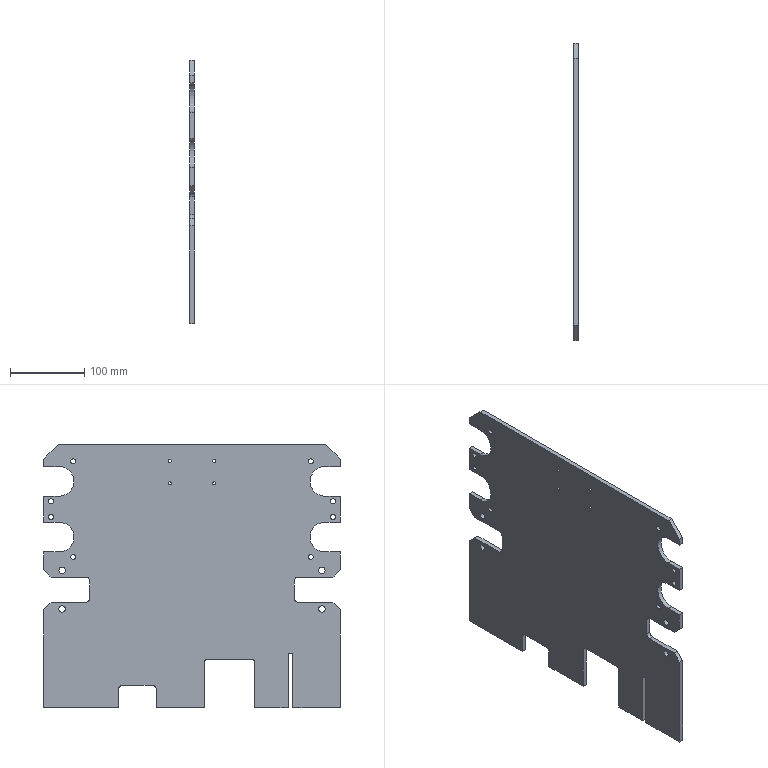Component | SolidWorks | THK-B1001RollerBracketLeft-1 | 1 solid | 88 faces | box 6 x 400 x 355 mm | volume 746106 mm3 | cylinder 44 | plane 44 | commonest cylinder face diameters 6.8 x16 4.2 x8 9 x8 40 x4 10 x4 8 x4 | material Q235A
build123d program:
from build123d import *

# Parameters (mm, degrees)
BOSS_EXTRUDE1_DEPTH      = 3
FILLET1_R                = 5
CHAMFER1_SIZE            = 10
M8_TAPPED_HOLE1_D        = 6.8
F_9_0_9_DIAMETER_HOLE1_D = 9
M5_TAPPED_HOLE2_D        = 4.2
CHAMFER2_SIZE            = 20
FILLET4_R                = 4


with BuildPart() as part:
    # Sketch1 → Boss-Extrude1 (new, symmetric)
    with BuildSketch(Plane(origin=(0, 0, 0), x_dir=(0, 0, -1), z_dir=(1, 0, 0))):
        with BuildLine():
            Line((-255, 200), (-113, 200))
            Line((-113, 200), (-113, 138))
            Line((-113, 138), (-79, 138))
            Line((-79, 138), (-79, 200))
            Line((-79, 200), (-45, 200))
            Line((-45, 200), (-45, 179))
            ThreePointArc((-45, 179), (-25, 159), (-5, 179))
            Line((-5, 179), (-5, 200))
            Line((-5, 200), (30, 200))
            Line((30, 200), (30, 179))
            ThreePointArc((30, 179), (50, 159), (70, 179))
            Line((70, 179), (70, 200))
            Line((70, 200), (100, 200))
            Line((100, 200), (100, -200))
            Line((100, -200), (70, -200))
            Line((70, -200), (70, -179))
            ThreePointArc((70, -179), (50, -159), (30, -179))
            Line((30, -179), (30, -200))
            Line((30, -200), (-5, -200))
            Line((-5, -200), (-5, -179))
            ThreePointArc((-5, -179), (-25, -159), (-45, -179))
            Line((-45, -179), (-45, -200))
            Line((-45, -200), (-79, -200))
            Line((-79, -200), (-79, -138))
            Line((-79, -138), (-113, -138))
            Line((-113, -138), (-113, -200))
            Line((-113, -200), (-255, -200))
            Line((-255, -200), (-255, -136))
            Line((-255, -136), (-182, -136))
            Line((-182, -136), (-182, -129.5))
            Line((-182, -129.5), (-255, -129.5))
            Line((-255, -129.5), (-255, -84.5))
            Line((-255, -84.5), (-190, -84.5))
            Line((-190, -84.5), (-190, -16.5))
            Line((-190, -16.5), (-255, -16.5))
            Line((-255, -16.5), (-255, 48.5))
            Line((-255, 48.5), (-225, 48.5))
            Line((-225, 48.5), (-225, 98.5))
            Line((-225, 98.5), (-255, 98.5))
            Line((-255, 98.5), (-255, 200))
        make_face()
    extrude(amount=BOSS_EXTRUDE1_DEPTH, both=True)

    # Fillet1
    fillet1_edges = [part.edges().sort_by_distance(p)[0] for p in [
        (0, 138, 113),
        (0, 138, 79),
        (0, -138, 79),
        (0, -138, 113),
    ]]
    fillet(fillet1_edges, radius=FILLET1_R)

    # Chamfer1
    chamfer1_edges = [part.edges().sort_by_distance(p)[0] for p in [
        (0, 200, 113),
        (0, 200, 79),
        (0, -200, 79),
        (0, -200, 113),
    ]]
    chamfer(chamfer1_edges, length=CHAMFER1_SIZE)

    # M8 Tapped Hole1 (through all)
    with Locations(Plane(origin=(3, 0, 0), x_dir=(0, 0, -1), z_dir=(1, 0, 0))):
        with Locations((2, 190), (23, 190), (-52, 160), (77, 160), (77, -160), (23, -190), (2, -190), (-52, -160)):
            Hole(M8_TAPPED_HOLE1_D / 2)

    # 9.0 _9_ Diameter Hole1 (through all)
    with Locations(Plane(origin=(3, 0, 0), x_dir=(0, 0, -1), z_dir=(1, 0, 0))):
        with Locations((-122, 175), (-70, 175), (-70, -175), (-122, -175)):
            Hole(F_9_0_9_DIAMETER_HOLE1_D / 2)

    # M5 Tapped Hole2 (through all)
    with Locations(Plane(origin=(3, 0, 0), x_dir=(0, 0, -1), z_dir=(1, 0, 0))):
        with Locations((47.5, 30), (77.5, 30), (77.5, -30), (47.5, -30)):
            Hole(M5_TAPPED_HOLE2_D / 2)

    # Chamfer2
    chamfer2_edges = [part.edges().sort_by_distance(p)[0] for p in [
        (0, 200, -100),
        (0, -200, -100),
    ]]
    chamfer(chamfer2_edges, length=CHAMFER2_SIZE)

    # Fillet4
    fillet4_edges = [part.edges().sort_by_distance(p)[0] for p in [
        (0, -84.5, 190),
        (0, -16.5, 190),
        (0, 48.5, 225),
        (0, 98.5, 225),
    ]]
    fillet(fillet4_edges, radius=FILLET4_R)


solid = part.part

# Placed as in the assembly
solid = solid.moved(Location((-130, 0, 0), (-180, 0, 180)))